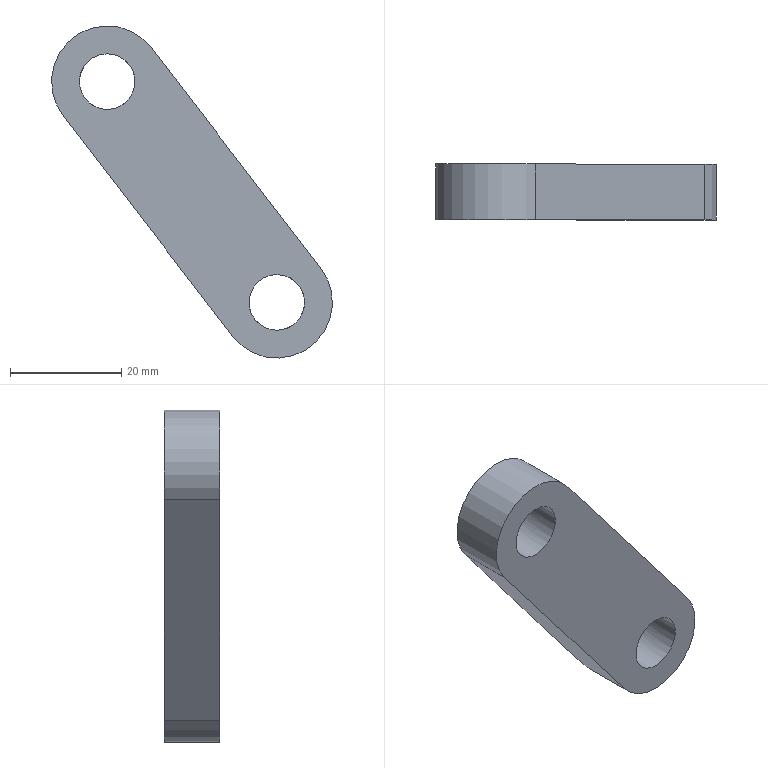Component | NX | 04 | 1 solid | 8 faces | box 50.46 x 10 x 59.65 mm | volume 11571 mm3 | cylinder 4 | plane 4 | commonest cylinder face diameters 20 x2 10 x2
STEP:
#1=CARTESIAN_POINT('',(0.,0.,0.));
#2=DIRECTION('',(0.,0.,1.));
#3=DIRECTION('',(1.,0.,0.));
#4=AXIS2_PLACEMENT_3D('',#1,#2,#3);
#5=CARTESIAN_POINT('',(212.473,25.,55.744));
#6=VERTEX_POINT('',#5);
#7=CARTESIAN_POINT('',(196.612,25.,43.561));
#8=VERTEX_POINT('',#7);
#9=CARTESIAN_POINT('',(204.543,25.,49.653));
#10=DIRECTION('',(0.,-1.,0.));
#11=DIRECTION('',(0.6091,0.,-0.7931));
#12=AXIS2_PLACEMENT_3D('',#9,#10,#11);
#13=CIRCLE('',#12,10.);
#14=CARTESIAN_POINT('',(204.543,15.,49.653));
#15=DIRECTION('',(0.,1.,0.));
#16=DIRECTION('',(0.7931,0.,0.6091));
#17=AXIS2_PLACEMENT_3D('',#14,#15,#16);
#18=CYLINDRICAL_SURFACE('',#17,10.);
#19=CARTESIAN_POINT('',(7.854,10.));
#20=DIRECTION('',(-1.,0.));
#21=VECTOR('',#20,1.);
#22=LINE('',#19,#21);
#23=(GEOMETRIC_REPRESENTATION_CONTEXT(2)PARAMETRIC_REPRESENTATION_CONTEXT()REPRESENTATION_CONTEXT('',''));
#24=DEFINITIONAL_REPRESENTATION('',(#22),#23);
#25=PCURVE('',#18,#24);
#26=CARTESIAN_POINT('',(204.543,25.,49.653));
#27=DIRECTION('',(0.,-1.,0.));
#28=DIRECTION('',(-0.7931,0.,-0.6091));
#29=AXIS2_PLACEMENT_3D('',#26,#27,#28);
#30=PLANE('',#29);
#31=CARTESIAN_POINT('',(0.,0.));
#32=DIRECTION('',(-0.,1.));
#33=AXIS2_PLACEMENT_2D('',#31,#32);
#34=CIRCLE('',#33,10.);
#35=(GEOMETRIC_REPRESENTATION_CONTEXT(2)PARAMETRIC_REPRESENTATION_CONTEXT()REPRESENTATION_CONTEXT('',''));
#36=DEFINITIONAL_REPRESENTATION('',(#34),#35);
#37=PCURVE('',#30,#36);
#38=SURFACE_CURVE('',#13,(#25,#37),.PCURVE_S1.);
#39=EDGE_CURVE('',#6,#8,#38,.T.);
#40=ORIENTED_EDGE('',*,*,#39,.T.);
#41=CARTESIAN_POINT('',(196.612,15.,43.561));
#42=VERTEX_POINT('',#41);
#43=CARTESIAN_POINT('',(196.612,15.,43.561));
#44=DIRECTION('',(0.,1.,0.));
#45=VECTOR('',#44,1.);
#46=LINE('',#43,#45);
#47=CARTESIAN_POINT('',(3.142,0.));
#48=DIRECTION('',(0.,1.));
#49=VECTOR('',#48,1.);
#50=LINE('',#47,#49);
#51=(GEOMETRIC_REPRESENTATION_CONTEXT(2)PARAMETRIC_REPRESENTATION_CONTEXT()REPRESENTATION_CONTEXT('',''));
#52=DEFINITIONAL_REPRESENTATION('',(#50),#51);
#53=PCURVE('',#18,#52);
#54=CARTESIAN_POINT('',(196.612,15.,43.561));
#55=DIRECTION('',(0.7931,0.,0.6091));
#56=DIRECTION('',(0.6091,0.,-0.7931));
#57=AXIS2_PLACEMENT_3D('',#54,#55,#56);
#58=PLANE('',#57);
#59=CARTESIAN_POINT('',(-0.,0.));
#60=DIRECTION('',(0.,1.));
#61=VECTOR('',#60,1.);
#62=LINE('',#59,#61);
#63=(GEOMETRIC_REPRESENTATION_CONTEXT(2)PARAMETRIC_REPRESENTATION_CONTEXT()REPRESENTATION_CONTEXT('',''));
#64=DEFINITIONAL_REPRESENTATION('',(#62),#63);
#65=PCURVE('',#58,#64);
#66=SURFACE_CURVE('',#46,(#53,#65),.PCURVE_S1.);
#67=EDGE_CURVE('',#42,#8,#66,.T.);
#68=ORIENTED_EDGE('',*,*,#67,.F.);
#69=CARTESIAN_POINT('',(212.473,15.,55.744));
#70=VERTEX_POINT('',#69);
#71=CARTESIAN_POINT('',(204.543,15.,49.653));
#72=DIRECTION('',(0.,-1.,0.));
#73=DIRECTION('',(0.6091,0.,-0.7931));
#74=AXIS2_PLACEMENT_3D('',#71,#72,#73);
#75=CIRCLE('',#74,10.);
#76=CARTESIAN_POINT('',(7.854,0.));
#77=DIRECTION('',(-1.,0.));
#78=VECTOR('',#77,1.);
#79=LINE('',#76,#78);
#80=(GEOMETRIC_REPRESENTATION_CONTEXT(2)PARAMETRIC_REPRESENTATION_CONTEXT()REPRESENTATION_CONTEXT('',''));
#81=DEFINITIONAL_REPRESENTATION('',(#79),#80);
#82=PCURVE('',#18,#81);
#83=CARTESIAN_POINT('',(204.543,15.,49.653));
#84=DIRECTION('',(0.,-1.,0.));
#85=DIRECTION('',(-0.7931,0.,-0.6091));
#86=AXIS2_PLACEMENT_3D('',#83,#84,#85);
#87=PLANE('',#86);
#88=CARTESIAN_POINT('',(0.,0.));
#89=DIRECTION('',(-0.,1.));
#90=AXIS2_PLACEMENT_2D('',#88,#89);
#91=CIRCLE('',#90,10.);
#92=(GEOMETRIC_REPRESENTATION_CONTEXT(2)PARAMETRIC_REPRESENTATION_CONTEXT()REPRESENTATION_CONTEXT('',''));
#93=DEFINITIONAL_REPRESENTATION('',(#91),#92);
#94=PCURVE('',#87,#93);
#95=SURFACE_CURVE('',#75,(#82,#94),.PCURVE_S1.);
#96=EDGE_CURVE('',#70,#42,#95,.T.);
#97=ORIENTED_EDGE('',*,*,#96,.F.);
#98=CARTESIAN_POINT('',(212.473,15.,55.744));
#99=DIRECTION('',(0.,1.,0.));
#100=VECTOR('',#99,1.);
#101=LINE('',#98,#100);
#102=CARTESIAN_POINT('',(6.283,0.));
#103=DIRECTION('',(0.,1.));
#104=VECTOR('',#103,1.);
#105=LINE('',#102,#104);
#106=(GEOMETRIC_REPRESENTATION_CONTEXT(2)PARAMETRIC_REPRESENTATION_CONTEXT()REPRESENTATION_CONTEXT('',''));
#107=DEFINITIONAL_REPRESENTATION('',(#105),#106);
#108=PCURVE('',#18,#107);
#109=CARTESIAN_POINT('',(242.931,15.,16.091));
#110=DIRECTION('',(-0.7931,0.,-0.6091));
#111=DIRECTION('',(-0.6091,0.,0.7931));
#112=AXIS2_PLACEMENT_3D('',#109,#110,#111);
#113=PLANE('',#112);
#114=CARTESIAN_POINT('',(50.,0.));
#115=DIRECTION('',(0.,1.));
#116=VECTOR('',#115,1.);
#117=LINE('',#114,#116);
#118=(GEOMETRIC_REPRESENTATION_CONTEXT(2)PARAMETRIC_REPRESENTATION_CONTEXT()REPRESENTATION_CONTEXT('',''));
#119=DEFINITIONAL_REPRESENTATION('',(#117),#118);
#120=PCURVE('',#113,#119);
#121=SURFACE_CURVE('',#101,(#108,#120),.PCURVE_S1.);
#122=EDGE_CURVE('',#70,#6,#121,.T.);
#123=ORIENTED_EDGE('',*,*,#122,.T.);
#124=EDGE_LOOP('',(#40,#68,#97,#123));
#125=FACE_BOUND('',#124,.T.);
#126=ADVANCED_FACE('',(#125),#18,.T.);
#127=CARTESIAN_POINT('',(227.069,25.,3.909));
#128=VERTEX_POINT('',#127);
#129=CARTESIAN_POINT('',(196.612,25.,43.561));
#130=DIRECTION('',(0.6091,0.,-0.7931));
#131=VECTOR('',#130,1.);
#132=LINE('',#129,#131);
#133=CARTESIAN_POINT('',(0.,10.));
#134=DIRECTION('',(1.,0.));
#135=VECTOR('',#134,1.);
#136=LINE('',#133,#135);
#137=(GEOMETRIC_REPRESENTATION_CONTEXT(2)PARAMETRIC_REPRESENTATION_CONTEXT()REPRESENTATION_CONTEXT('',''));
#138=DEFINITIONAL_REPRESENTATION('',(#136),#137);
#139=PCURVE('',#58,#138);
#140=CARTESIAN_POINT('',(10.,0.));
#141=DIRECTION('',(0.,1.));
#142=VECTOR('',#141,1.);
#143=LINE('',#140,#142);
#144=(GEOMETRIC_REPRESENTATION_CONTEXT(2)PARAMETRIC_REPRESENTATION_CONTEXT()REPRESENTATION_CONTEXT('',''));
#145=DEFINITIONAL_REPRESENTATION('',(#143),#144);
#146=PCURVE('',#30,#145);
#147=SURFACE_CURVE('',#132,(#139,#146),.PCURVE_S1.);
#148=EDGE_CURVE('',#8,#128,#147,.T.);
#149=ORIENTED_EDGE('',*,*,#148,.T.);
#150=CARTESIAN_POINT('',(227.069,15.,3.909));
#151=VERTEX_POINT('',#150);
#152=CARTESIAN_POINT('',(227.069,15.,3.909));
#153=DIRECTION('',(0.,1.,0.));
#154=VECTOR('',#153,1.);
#155=LINE('',#152,#154);
#156=CARTESIAN_POINT('',(50.,0.));
#157=DIRECTION('',(0.,1.));
#158=VECTOR('',#157,1.);
#159=LINE('',#156,#158);
#160=(GEOMETRIC_REPRESENTATION_CONTEXT(2)PARAMETRIC_REPRESENTATION_CONTEXT()REPRESENTATION_CONTEXT('',''));
#161=DEFINITIONAL_REPRESENTATION('',(#159),#160);
#162=PCURVE('',#58,#161);
#163=CARTESIAN_POINT('',(235.,15.,10.));
#164=DIRECTION('',(0.,1.,0.));
#165=DIRECTION('',(0.7931,0.,0.6091));
#166=AXIS2_PLACEMENT_3D('',#163,#164,#165);
#167=CYLINDRICAL_SURFACE('',#166,10.);
#168=CARTESIAN_POINT('',(3.142,0.));
#169=DIRECTION('',(0.,1.));
#170=VECTOR('',#169,1.);
#171=LINE('',#168,#170);
#172=(GEOMETRIC_REPRESENTATION_CONTEXT(2)PARAMETRIC_REPRESENTATION_CONTEXT()REPRESENTATION_CONTEXT('',''));
#173=DEFINITIONAL_REPRESENTATION('',(#171),#172);
#174=PCURVE('',#167,#173);
#175=SURFACE_CURVE('',#155,(#162,#174),.PCURVE_S1.);
#176=EDGE_CURVE('',#151,#128,#175,.T.);
#177=ORIENTED_EDGE('',*,*,#176,.F.);
#178=CARTESIAN_POINT('',(196.612,15.,43.561));
#179=DIRECTION('',(0.6091,0.,-0.7931));
#180=VECTOR('',#179,1.);
#181=LINE('',#178,#180);
#182=CARTESIAN_POINT('',(0.,0.));
#183=DIRECTION('',(1.,0.));
#184=VECTOR('',#183,1.);
#185=LINE('',#182,#184);
#186=(GEOMETRIC_REPRESENTATION_CONTEXT(2)PARAMETRIC_REPRESENTATION_CONTEXT()REPRESENTATION_CONTEXT('',''));
#187=DEFINITIONAL_REPRESENTATION('',(#185),#186);
#188=PCURVE('',#58,#187);
#189=CARTESIAN_POINT('',(10.,0.));
#190=DIRECTION('',(0.,1.));
#191=VECTOR('',#190,1.);
#192=LINE('',#189,#191);
#193=(GEOMETRIC_REPRESENTATION_CONTEXT(2)PARAMETRIC_REPRESENTATION_CONTEXT()REPRESENTATION_CONTEXT('',''));
#194=DEFINITIONAL_REPRESENTATION('',(#192),#193);
#195=PCURVE('',#87,#194);
#196=SURFACE_CURVE('',#181,(#188,#195),.PCURVE_S1.);
#197=EDGE_CURVE('',#42,#151,#196,.T.);
#198=ORIENTED_EDGE('',*,*,#197,.F.);
#199=ORIENTED_EDGE('',*,*,#67,.T.);
#200=EDGE_LOOP('',(#149,#177,#198,#199));
#201=FACE_BOUND('',#200,.T.);
#202=ADVANCED_FACE('',(#201),#58,.F.);
#203=CARTESIAN_POINT('',(242.931,25.,16.091));
#204=VERTEX_POINT('',#203);
#205=CARTESIAN_POINT('',(235.,25.,10.));
#206=DIRECTION('',(0.,-1.,0.));
#207=DIRECTION('',(0.6091,0.,-0.7931));
#208=AXIS2_PLACEMENT_3D('',#205,#206,#207);
#209=CIRCLE('',#208,10.);
#210=CARTESIAN_POINT('',(7.854,10.));
#211=DIRECTION('',(-1.,0.));
#212=VECTOR('',#211,1.);
#213=LINE('',#210,#212);
#214=(GEOMETRIC_REPRESENTATION_CONTEXT(2)PARAMETRIC_REPRESENTATION_CONTEXT()REPRESENTATION_CONTEXT('',''));
#215=DEFINITIONAL_REPRESENTATION('',(#213),#214);
#216=PCURVE('',#167,#215);
#217=CARTESIAN_POINT('',(-0.,50.));
#218=DIRECTION('',(-0.,1.));
#219=AXIS2_PLACEMENT_2D('',#217,#218);
#220=CIRCLE('',#219,10.);
#221=(GEOMETRIC_REPRESENTATION_CONTEXT(2)PARAMETRIC_REPRESENTATION_CONTEXT()REPRESENTATION_CONTEXT('',''));
#222=DEFINITIONAL_REPRESENTATION('',(#220),#221);
#223=PCURVE('',#30,#222);
#224=SURFACE_CURVE('',#209,(#216,#223),.PCURVE_S1.);
#225=EDGE_CURVE('',#128,#204,#224,.T.);
#226=ORIENTED_EDGE('',*,*,#225,.T.);
#227=CARTESIAN_POINT('',(242.931,15.,16.091));
#228=VERTEX_POINT('',#227);
#229=CARTESIAN_POINT('',(242.931,15.,16.091));
#230=DIRECTION('',(0.,1.,0.));
#231=VECTOR('',#230,1.);
#232=LINE('',#229,#231);
#233=CARTESIAN_POINT('',(0.,0.));
#234=DIRECTION('',(0.,1.));
#235=VECTOR('',#234,1.);
#236=LINE('',#233,#235);
#237=(GEOMETRIC_REPRESENTATION_CONTEXT(2)PARAMETRIC_REPRESENTATION_CONTEXT()REPRESENTATION_CONTEXT('',''));
#238=DEFINITIONAL_REPRESENTATION('',(#236),#237);
#239=PCURVE('',#167,#238);
#240=CARTESIAN_POINT('',(0.,0.));
#241=DIRECTION('',(0.,1.));
#242=VECTOR('',#241,1.);
#243=LINE('',#240,#242);
#244=(GEOMETRIC_REPRESENTATION_CONTEXT(2)PARAMETRIC_REPRESENTATION_CONTEXT()REPRESENTATION_CONTEXT('',''));
#245=DEFINITIONAL_REPRESENTATION('',(#243),#244);
#246=PCURVE('',#113,#245);
#247=SURFACE_CURVE('',#232,(#239,#246),.PCURVE_S1.);
#248=EDGE_CURVE('',#228,#204,#247,.T.);
#249=ORIENTED_EDGE('',*,*,#248,.F.);
#250=CARTESIAN_POINT('',(235.,15.,10.));
#251=DIRECTION('',(0.,-1.,0.));
#252=DIRECTION('',(0.6091,0.,-0.7931));
#253=AXIS2_PLACEMENT_3D('',#250,#251,#252);
#254=CIRCLE('',#253,10.);
#255=CARTESIAN_POINT('',(7.854,0.));
#256=DIRECTION('',(-1.,0.));
#257=VECTOR('',#256,1.);
#258=LINE('',#255,#257);
#259=(GEOMETRIC_REPRESENTATION_CONTEXT(2)PARAMETRIC_REPRESENTATION_CONTEXT()REPRESENTATION_CONTEXT('',''));
#260=DEFINITIONAL_REPRESENTATION('',(#258),#259);
#261=PCURVE('',#167,#260);
#262=CARTESIAN_POINT('',(-0.,50.));
#263=DIRECTION('',(-0.,1.));
#264=AXIS2_PLACEMENT_2D('',#262,#263);
#265=CIRCLE('',#264,10.);
#266=(GEOMETRIC_REPRESENTATION_CONTEXT(2)PARAMETRIC_REPRESENTATION_CONTEXT()REPRESENTATION_CONTEXT('',''));
#267=DEFINITIONAL_REPRESENTATION('',(#265),#266);
#268=PCURVE('',#87,#267);
#269=SURFACE_CURVE('',#254,(#261,#268),.PCURVE_S1.);
#270=EDGE_CURVE('',#151,#228,#269,.T.);
#271=ORIENTED_EDGE('',*,*,#270,.F.);
#272=ORIENTED_EDGE('',*,*,#176,.T.);
#273=EDGE_LOOP('',(#226,#249,#271,#272));
#274=FACE_BOUND('',#273,.T.);
#275=ADVANCED_FACE('',(#274),#167,.T.);
#276=CARTESIAN_POINT('',(242.931,25.,16.091));
#277=DIRECTION('',(-0.6091,0.,0.7931));
#278=VECTOR('',#277,1.);
#279=LINE('',#276,#278);
#280=CARTESIAN_POINT('',(0.,10.));
#281=DIRECTION('',(1.,0.));
#282=VECTOR('',#281,1.);
#283=LINE('',#280,#282);
#284=(GEOMETRIC_REPRESENTATION_CONTEXT(2)PARAMETRIC_REPRESENTATION_CONTEXT()REPRESENTATION_CONTEXT('',''));
#285=DEFINITIONAL_REPRESENTATION('',(#283),#284);
#286=PCURVE('',#113,#285);
#287=CARTESIAN_POINT('',(-10.,50.));
#288=DIRECTION('',(0.,-1.));
#289=VECTOR('',#288,1.);
#290=LINE('',#287,#289);
#291=(GEOMETRIC_REPRESENTATION_CONTEXT(2)PARAMETRIC_REPRESENTATION_CONTEXT()REPRESENTATION_CONTEXT('',''));
#292=DEFINITIONAL_REPRESENTATION('',(#290),#291);
#293=PCURVE('',#30,#292);
#294=SURFACE_CURVE('',#279,(#286,#293),.PCURVE_S1.);
#295=EDGE_CURVE('',#204,#6,#294,.T.);
#296=ORIENTED_EDGE('',*,*,#295,.T.);
#297=ORIENTED_EDGE('',*,*,#122,.F.);
#298=CARTESIAN_POINT('',(242.931,15.,16.091));
#299=DIRECTION('',(-0.6091,0.,0.7931));
#300=VECTOR('',#299,1.);
#301=LINE('',#298,#300);
#302=CARTESIAN_POINT('',(0.,0.));
#303=DIRECTION('',(1.,0.));
#304=VECTOR('',#303,1.);
#305=LINE('',#302,#304);
#306=(GEOMETRIC_REPRESENTATION_CONTEXT(2)PARAMETRIC_REPRESENTATION_CONTEXT()REPRESENTATION_CONTEXT('',''));
#307=DEFINITIONAL_REPRESENTATION('',(#305),#306);
#308=PCURVE('',#113,#307);
#309=CARTESIAN_POINT('',(-10.,50.));
#310=DIRECTION('',(0.,-1.));
#311=VECTOR('',#310,1.);
#312=LINE('',#309,#311);
#313=(GEOMETRIC_REPRESENTATION_CONTEXT(2)PARAMETRIC_REPRESENTATION_CONTEXT()REPRESENTATION_CONTEXT('',''));
#314=DEFINITIONAL_REPRESENTATION('',(#312),#313);
#315=PCURVE('',#87,#314);
#316=SURFACE_CURVE('',#301,(#308,#315),.PCURVE_S1.);
#317=EDGE_CURVE('',#228,#70,#316,.T.);
#318=ORIENTED_EDGE('',*,*,#317,.F.);
#319=ORIENTED_EDGE('',*,*,#248,.T.);
#320=EDGE_LOOP('',(#296,#297,#318,#319));
#321=FACE_BOUND('',#320,.T.);
#322=ADVANCED_FACE('',(#321),#113,.F.);
#323=CARTESIAN_POINT('',(238.046,15.,6.035));
#324=VERTEX_POINT('',#323);
#325=CARTESIAN_POINT('',(231.035,15.,6.954));
#326=VERTEX_POINT('',#325);
#327=CARTESIAN_POINT('',(235.,15.,10.));
#328=DIRECTION('',(0.,-1.,0.));
#329=DIRECTION('',(0.6091,0.,-0.7931));
#330=AXIS2_PLACEMENT_3D('',#327,#328,#329);
#331=CIRCLE('',#330,5.);
#332=CARTESIAN_POINT('',(-0.,50.));
#333=DIRECTION('',(0.,1.));
#334=AXIS2_PLACEMENT_2D('',#332,#333);
#335=CIRCLE('',#334,5.);
#336=(GEOMETRIC_REPRESENTATION_CONTEXT(2)PARAMETRIC_REPRESENTATION_CONTEXT()REPRESENTATION_CONTEXT('',''));
#337=DEFINITIONAL_REPRESENTATION('',(#335),#336);
#338=PCURVE('',#87,#337);
#339=CARTESIAN_POINT('',(235.,35.,10.));
#340=DIRECTION('',(0.,-1.,0.));
#341=DIRECTION('',(-0.7931,0.,-0.6091));
#342=AXIS2_PLACEMENT_3D('',#339,#340,#341);
#343=CYLINDRICAL_SURFACE('',#342,5.);
#344=CARTESIAN_POINT('',(1.571,20.));
#345=DIRECTION('',(1.,0.));
#346=VECTOR('',#345,1.);
#347=LINE('',#344,#346);
#348=(GEOMETRIC_REPRESENTATION_CONTEXT(2)PARAMETRIC_REPRESENTATION_CONTEXT()REPRESENTATION_CONTEXT('',''));
#349=DEFINITIONAL_REPRESENTATION('',(#347),#348);
#350=PCURVE('',#343,#349);
#351=SURFACE_CURVE('',#331,(#338,#350),.PCURVE_S1.);
#352=EDGE_CURVE('',#324,#326,#351,.T.);
#353=ORIENTED_EDGE('',*,*,#352,.F.);
#354=CARTESIAN_POINT('',(235.,15.,10.));
#355=DIRECTION('',(0.,-1.,0.));
#356=DIRECTION('',(0.6091,0.,-0.7931));
#357=AXIS2_PLACEMENT_3D('',#354,#355,#356);
#358=CIRCLE('',#357,5.);
#359=CARTESIAN_POINT('',(-0.,50.));
#360=DIRECTION('',(0.,1.));
#361=AXIS2_PLACEMENT_2D('',#359,#360);
#362=CIRCLE('',#361,5.);
#363=(GEOMETRIC_REPRESENTATION_CONTEXT(2)PARAMETRIC_REPRESENTATION_CONTEXT()REPRESENTATION_CONTEXT('',''));
#364=DEFINITIONAL_REPRESENTATION('',(#362),#363);
#365=PCURVE('',#87,#364);
#366=CARTESIAN_POINT('',(-4.712,20.));
#367=DIRECTION('',(1.,0.));
#368=VECTOR('',#367,1.);
#369=LINE('',#366,#368);
#370=(GEOMETRIC_REPRESENTATION_CONTEXT(2)PARAMETRIC_REPRESENTATION_CONTEXT()REPRESENTATION_CONTEXT('',''));
#371=DEFINITIONAL_REPRESENTATION('',(#369),#370);
#372=PCURVE('',#343,#371);
#373=SURFACE_CURVE('',#358,(#365,#372),.PCURVE_S1.);
#374=EDGE_CURVE('',#326,#324,#373,.T.);
#375=ORIENTED_EDGE('',*,*,#374,.F.);
#376=EDGE_LOOP('',(#353,#375));
#377=FACE_BOUND('',#376,.T.);
#378=CARTESIAN_POINT('',(207.588,15.,45.688));
#379=VERTEX_POINT('',#378);
#380=CARTESIAN_POINT('',(200.577,15.,46.607));
#381=VERTEX_POINT('',#380);
#382=CARTESIAN_POINT('',(204.543,15.,49.653));
#383=DIRECTION('',(0.,-1.,0.));
#384=DIRECTION('',(0.6091,0.,-0.7931));
#385=AXIS2_PLACEMENT_3D('',#382,#383,#384);
#386=CIRCLE('',#385,5.);
#387=CARTESIAN_POINT('',(0.,0.));
#388=DIRECTION('',(0.,1.));
#389=AXIS2_PLACEMENT_2D('',#387,#388);
#390=CIRCLE('',#389,5.);
#391=(GEOMETRIC_REPRESENTATION_CONTEXT(2)PARAMETRIC_REPRESENTATION_CONTEXT()REPRESENTATION_CONTEXT('',''));
#392=DEFINITIONAL_REPRESENTATION('',(#390),#391);
#393=PCURVE('',#87,#392);
#394=CARTESIAN_POINT('',(204.543,35.,49.653));
#395=DIRECTION('',(0.,-1.,0.));
#396=DIRECTION('',(-0.7931,0.,-0.6091));
#397=AXIS2_PLACEMENT_3D('',#394,#395,#396);
#398=CYLINDRICAL_SURFACE('',#397,5.);
#399=CARTESIAN_POINT('',(1.571,20.));
#400=DIRECTION('',(1.,0.));
#401=VECTOR('',#400,1.);
#402=LINE('',#399,#401);
#403=(GEOMETRIC_REPRESENTATION_CONTEXT(2)PARAMETRIC_REPRESENTATION_CONTEXT()REPRESENTATION_CONTEXT('',''));
#404=DEFINITIONAL_REPRESENTATION('',(#402),#403);
#405=PCURVE('',#398,#404);
#406=SURFACE_CURVE('',#386,(#393,#405),.PCURVE_S1.);
#407=EDGE_CURVE('',#379,#381,#406,.T.);
#408=ORIENTED_EDGE('',*,*,#407,.F.);
#409=CARTESIAN_POINT('',(204.543,15.,49.653));
#410=DIRECTION('',(0.,-1.,0.));
#411=DIRECTION('',(0.6091,0.,-0.7931));
#412=AXIS2_PLACEMENT_3D('',#409,#410,#411);
#413=CIRCLE('',#412,5.);
#414=CARTESIAN_POINT('',(0.,0.));
#415=DIRECTION('',(0.,1.));
#416=AXIS2_PLACEMENT_2D('',#414,#415);
#417=CIRCLE('',#416,5.);
#418=(GEOMETRIC_REPRESENTATION_CONTEXT(2)PARAMETRIC_REPRESENTATION_CONTEXT()REPRESENTATION_CONTEXT('',''));
#419=DEFINITIONAL_REPRESENTATION('',(#417),#418);
#420=PCURVE('',#87,#419);
#421=CARTESIAN_POINT('',(-4.712,20.));
#422=DIRECTION('',(1.,0.));
#423=VECTOR('',#422,1.);
#424=LINE('',#421,#423);
#425=(GEOMETRIC_REPRESENTATION_CONTEXT(2)PARAMETRIC_REPRESENTATION_CONTEXT()REPRESENTATION_CONTEXT('',''));
#426=DEFINITIONAL_REPRESENTATION('',(#424),#425);
#427=PCURVE('',#398,#426);
#428=SURFACE_CURVE('',#413,(#420,#427),.PCURVE_S1.);
#429=EDGE_CURVE('',#381,#379,#428,.T.);
#430=ORIENTED_EDGE('',*,*,#429,.F.);
#431=EDGE_LOOP('',(#408,#430));
#432=FACE_BOUND('',#431,.T.);
#433=ORIENTED_EDGE('',*,*,#96,.T.);
#434=ORIENTED_EDGE('',*,*,#197,.T.);
#435=ORIENTED_EDGE('',*,*,#270,.T.);
#436=ORIENTED_EDGE('',*,*,#317,.T.);
#437=EDGE_LOOP('',(#433,#434,#435,#436));
#438=FACE_BOUND('',#437,.T.);
#439=ADVANCED_FACE('',(#377,#432,#438),#87,.T.);
#440=CARTESIAN_POINT('',(231.035,25.,6.954));
#441=VERTEX_POINT('',#440);
#442=CARTESIAN_POINT('',(235.,25.,10.));
#443=DIRECTION('',(0.,-1.,0.));
#444=DIRECTION('',(-0.7931,0.,-0.6091));
#445=AXIS2_PLACEMENT_3D('',#442,#443,#444);
#446=CIRCLE('',#445,5.);
#447=CARTESIAN_POINT('',(-0.,50.));
#448=DIRECTION('',(1.,-0.));
#449=AXIS2_PLACEMENT_2D('',#447,#448);
#450=CIRCLE('',#449,5.);
#451=(GEOMETRIC_REPRESENTATION_CONTEXT(2)PARAMETRIC_REPRESENTATION_CONTEXT()REPRESENTATION_CONTEXT('',''));
#452=DEFINITIONAL_REPRESENTATION('',(#450),#451);
#453=PCURVE('',#30,#452);
#454=CARTESIAN_POINT('',(0.,10.));
#455=DIRECTION('',(1.,0.));
#456=VECTOR('',#455,1.);
#457=LINE('',#454,#456);
#458=(GEOMETRIC_REPRESENTATION_CONTEXT(2)PARAMETRIC_REPRESENTATION_CONTEXT()REPRESENTATION_CONTEXT('',''));
#459=DEFINITIONAL_REPRESENTATION('',(#457),#458);
#460=PCURVE('',#343,#459);
#461=SURFACE_CURVE('',#446,(#453,#460),.PCURVE_S1.);
#462=EDGE_CURVE('',#441,#441,#461,.T.);
#463=ORIENTED_EDGE('',*,*,#462,.T.);
#464=EDGE_LOOP('',(#463));
#465=FACE_BOUND('',#464,.T.);
#466=CARTESIAN_POINT('',(200.577,25.,46.607));
#467=VERTEX_POINT('',#466);
#468=CARTESIAN_POINT('',(204.543,25.,49.653));
#469=DIRECTION('',(0.,-1.,0.));
#470=DIRECTION('',(-0.7931,0.,-0.6091));
#471=AXIS2_PLACEMENT_3D('',#468,#469,#470);
#472=CIRCLE('',#471,5.);
#473=CARTESIAN_POINT('',(0.,0.));
#474=DIRECTION('',(1.,-0.));
#475=AXIS2_PLACEMENT_2D('',#473,#474);
#476=CIRCLE('',#475,5.);
#477=(GEOMETRIC_REPRESENTATION_CONTEXT(2)PARAMETRIC_REPRESENTATION_CONTEXT()REPRESENTATION_CONTEXT('',''));
#478=DEFINITIONAL_REPRESENTATION('',(#476),#477);
#479=PCURVE('',#30,#478);
#480=CARTESIAN_POINT('',(0.,10.));
#481=DIRECTION('',(1.,0.));
#482=VECTOR('',#481,1.);
#483=LINE('',#480,#482);
#484=(GEOMETRIC_REPRESENTATION_CONTEXT(2)PARAMETRIC_REPRESENTATION_CONTEXT()REPRESENTATION_CONTEXT('',''));
#485=DEFINITIONAL_REPRESENTATION('',(#483),#484);
#486=PCURVE('',#398,#485);
#487=SURFACE_CURVE('',#472,(#479,#486),.PCURVE_S1.);
#488=EDGE_CURVE('',#467,#467,#487,.T.);
#489=ORIENTED_EDGE('',*,*,#488,.T.);
#490=EDGE_LOOP('',(#489));
#491=FACE_BOUND('',#490,.T.);
#492=ORIENTED_EDGE('',*,*,#39,.F.);
#493=ORIENTED_EDGE('',*,*,#295,.F.);
#494=ORIENTED_EDGE('',*,*,#225,.F.);
#495=ORIENTED_EDGE('',*,*,#148,.F.);
#496=EDGE_LOOP('',(#492,#493,#494,#495));
#497=FACE_BOUND('',#496,.T.);
#498=ADVANCED_FACE('',(#465,#491,#497),#30,.F.);
#499=ORIENTED_EDGE('',*,*,#429,.F.);
#500=CARTESIAN_POINT('',(200.577,25.,46.607));
#501=CARTESIAN_POINT('',(200.577,15.,46.607));
#502=B_SPLINE_CURVE_WITH_KNOTS('',1,(#500,#501),.UNSPECIFIED.,.F.,.F.,(2,2),(10.,20.),.PIECEWISE_BEZIER_KNOTS.);
#503=CARTESIAN_POINT('',(0.,0.));
#504=DIRECTION('',(0.,1.));
#505=VECTOR('',#504,1.);
#506=LINE('',#503,#505);
#507=(GEOMETRIC_REPRESENTATION_CONTEXT(2)PARAMETRIC_REPRESENTATION_CONTEXT()REPRESENTATION_CONTEXT('',''));
#508=DEFINITIONAL_REPRESENTATION('',(#506),#507);
#509=PCURVE('',#398,#508);
#510=CARTESIAN_POINT('',(6.283,0.));
#511=DIRECTION('',(0.,1.));
#512=VECTOR('',#511,1.);
#513=LINE('',#510,#512);
#514=(GEOMETRIC_REPRESENTATION_CONTEXT(2)PARAMETRIC_REPRESENTATION_CONTEXT()REPRESENTATION_CONTEXT('',''));
#515=DEFINITIONAL_REPRESENTATION('',(#513),#514);
#516=PCURVE('',#398,#515);
#517=SEAM_CURVE('',#502,(#509,#516),.PCURVE_S1.);
#518=EDGE_CURVE('',#467,#381,#517,.T.);
#519=ORIENTED_EDGE('',*,*,#518,.F.);
#520=ORIENTED_EDGE('',*,*,#488,.T.);
#521=ORIENTED_EDGE('',*,*,#518,.T.);
#522=ORIENTED_EDGE('',*,*,#407,.F.);
#523=EDGE_LOOP('',(#499,#519,#520,#521,#522));
#524=FACE_BOUND('',#523,.F.);
#525=ADVANCED_FACE('',(#524),#398,.F.);
#526=ORIENTED_EDGE('',*,*,#374,.F.);
#527=CARTESIAN_POINT('',(231.035,25.,6.954));
#528=CARTESIAN_POINT('',(231.035,15.,6.954));
#529=B_SPLINE_CURVE_WITH_KNOTS('',1,(#527,#528),.UNSPECIFIED.,.F.,.F.,(2,2),(10.,20.),.PIECEWISE_BEZIER_KNOTS.);
#530=CARTESIAN_POINT('',(0.,0.));
#531=DIRECTION('',(0.,1.));
#532=VECTOR('',#531,1.);
#533=LINE('',#530,#532);
#534=(GEOMETRIC_REPRESENTATION_CONTEXT(2)PARAMETRIC_REPRESENTATION_CONTEXT()REPRESENTATION_CONTEXT('',''));
#535=DEFINITIONAL_REPRESENTATION('',(#533),#534);
#536=PCURVE('',#343,#535);
#537=CARTESIAN_POINT('',(6.283,0.));
#538=DIRECTION('',(0.,1.));
#539=VECTOR('',#538,1.);
#540=LINE('',#537,#539);
#541=(GEOMETRIC_REPRESENTATION_CONTEXT(2)PARAMETRIC_REPRESENTATION_CONTEXT()REPRESENTATION_CONTEXT('',''));
#542=DEFINITIONAL_REPRESENTATION('',(#540),#541);
#543=PCURVE('',#343,#542);
#544=SEAM_CURVE('',#529,(#536,#543),.PCURVE_S1.);
#545=EDGE_CURVE('',#441,#326,#544,.T.);
#546=ORIENTED_EDGE('',*,*,#545,.F.);
#547=ORIENTED_EDGE('',*,*,#462,.T.);
#548=ORIENTED_EDGE('',*,*,#545,.T.);
#549=ORIENTED_EDGE('',*,*,#352,.F.);
#550=EDGE_LOOP('',(#526,#546,#547,#548,#549));
#551=FACE_BOUND('',#550,.F.);
#552=ADVANCED_FACE('',(#551),#343,.F.);
#553=CLOSED_SHELL('',(#126,#202,#275,#322,#439,#498,#525,#552));
#554=MANIFOLD_SOLID_BREP('',#553);
#555=(LENGTH_UNIT()NAMED_UNIT(*)SI_UNIT(.MILLI.,.METRE.));
#556=UNCERTAINTY_MEASURE_WITH_UNIT(LENGTH_MEASURE(0.000002),#555,'','');
#557=(NAMED_UNIT(*)PLANE_ANGLE_UNIT()SI_UNIT($,.RADIAN.));
#558=(NAMED_UNIT(*)SI_UNIT($,.STERADIAN.)SOLID_ANGLE_UNIT());
#559=(GEOMETRIC_REPRESENTATION_CONTEXT(3)GLOBAL_UNCERTAINTY_ASSIGNED_CONTEXT((#556))GLOBAL_UNIT_ASSIGNED_CONTEXT((#555,#557,#558))REPRESENTATION_CONTEXT('',''));
#560=ADVANCED_BREP_SHAPE_REPRESENTATION('',(#4,#554),#559);